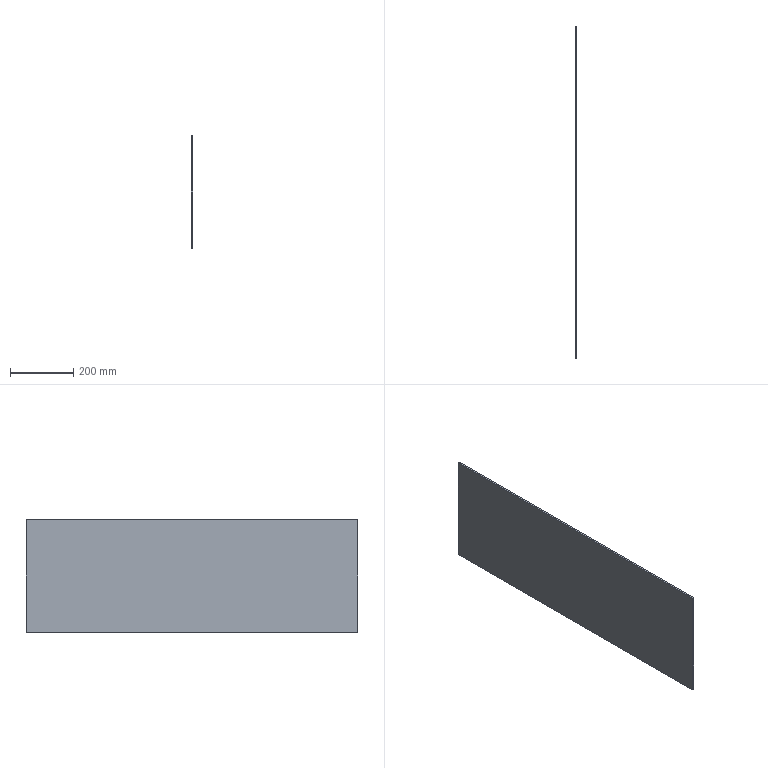Component | SolidWorks | BrownAcrylicPlate-5_BrownAcrylicPlate-2-2 | 1 solid | 6 faces | box 6 x 1049.15 x 355 mm | volume 2234689 mm3 | plane 6
STEP:
#1=CARTESIAN_POINT('',(-0.4379,39.232,-55.138));
#2=VERTEX_POINT('',#1);
#3=CARTESIAN_POINT('',(-0.4379,39.232,-69.114));
#4=VERTEX_POINT('',#3);
#5=CARTESIAN_POINT('',(-0.4379,39.232,-70.886));
#6=DIRECTION('',(-0.,0.,-1.));
#7=VECTOR('',#6,39.37);
#8=LINE('',#5,#7);
#9=EDGE_CURVE('',#2,#4,#8,.T.);
#10=ORIENTED_EDGE('',*,*,#9,.T.);
#11=CARTESIAN_POINT('',(-0.4379,80.537,-69.114));
#12=VERTEX_POINT('',#11);
#13=CARTESIAN_POINT('',(-0.4379,80.537,-69.114));
#14=DIRECTION('',(0.,1.,0.));
#15=VECTOR('',#14,39.37);
#16=LINE('',#13,#15);
#17=EDGE_CURVE('',#4,#12,#16,.T.);
#18=ORIENTED_EDGE('',*,*,#17,.T.);
#19=CARTESIAN_POINT('',(-0.4379,80.537,-55.138));
#20=VERTEX_POINT('',#19);
#21=CARTESIAN_POINT('',(-0.4379,80.537,-70.886));
#22=DIRECTION('',(0.,-0.,1.));
#23=VECTOR('',#22,39.37);
#24=LINE('',#21,#23);
#25=EDGE_CURVE('',#12,#20,#24,.T.);
#26=ORIENTED_EDGE('',*,*,#25,.T.);
#27=CARTESIAN_POINT('',(-0.4379,80.537,-55.138));
#28=DIRECTION('',(-0.,-1.,-0.));
#29=VECTOR('',#28,39.37);
#30=LINE('',#27,#29);
#31=EDGE_CURVE('',#20,#2,#30,.T.);
#32=ORIENTED_EDGE('',*,*,#31,.T.);
#33=EDGE_LOOP('',(#10,#18,#26,#32));
#34=FACE_OUTER_BOUND('',#33,.T.);
#35=CARTESIAN_POINT('',(-0.4379,69.711,-63.012));
#36=DIRECTION('',(1.,-0.,-0.));
#37=DIRECTION('',(0.,1.,0.));
#38=AXIS2_PLACEMENT_3D('',#35,#36,#37);
#39=PLANE('',#38);
#40=ADVANCED_FACE('',(#34),#39,.T.);
#41=CARTESIAN_POINT('',(-0.6741,39.232,-69.114));
#42=VERTEX_POINT('',#41);
#43=CARTESIAN_POINT('',(-0.6741,80.537,-69.114));
#44=VERTEX_POINT('',#43);
#45=CARTESIAN_POINT('',(-0.6741,69.711,-69.114));
#46=DIRECTION('',(0.,1.,0.));
#47=VECTOR('',#46,39.37);
#48=LINE('',#45,#47);
#49=EDGE_CURVE('',#42,#44,#48,.T.);
#50=ORIENTED_EDGE('',*,*,#49,.F.);
#51=CARTESIAN_POINT('',(-0.6741,39.232,-55.138));
#52=VERTEX_POINT('',#51);
#53=CARTESIAN_POINT('',(-0.6741,39.232,-63.012));
#54=DIRECTION('',(-0.,0.,-1.));
#55=VECTOR('',#54,39.37);
#56=LINE('',#53,#55);
#57=EDGE_CURVE('',#52,#42,#56,.T.);
#58=ORIENTED_EDGE('',*,*,#57,.F.);
#59=CARTESIAN_POINT('',(-0.6741,80.537,-55.138));
#60=VERTEX_POINT('',#59);
#61=CARTESIAN_POINT('',(-0.6741,69.711,-55.138));
#62=DIRECTION('',(-0.,-1.,-0.));
#63=VECTOR('',#62,39.37);
#64=LINE('',#61,#63);
#65=EDGE_CURVE('',#60,#52,#64,.T.);
#66=ORIENTED_EDGE('',*,*,#65,.F.);
#67=CARTESIAN_POINT('',(-0.6741,80.537,-63.012));
#68=DIRECTION('',(0.,-0.,1.));
#69=VECTOR('',#68,39.37);
#70=LINE('',#67,#69);
#71=EDGE_CURVE('',#44,#60,#70,.T.);
#72=ORIENTED_EDGE('',*,*,#71,.F.);
#73=EDGE_LOOP('',(#50,#58,#66,#72));
#74=FACE_OUTER_BOUND('',#73,.T.);
#75=CARTESIAN_POINT('',(-0.6741,69.711,-63.012));
#76=DIRECTION('',(1.,-0.,-0.));
#77=DIRECTION('',(0.,1.,0.));
#78=AXIS2_PLACEMENT_3D('',#75,#76,#77);
#79=PLANE('',#78);
#80=ADVANCED_FACE('',(#74),#79,.F.);
#81=ORIENTED_EDGE('',*,*,#71,.T.);
#82=CARTESIAN_POINT('',(-0.6741,80.537,-55.138));
#83=DIRECTION('',(1.,-0.,-0.));
#84=VECTOR('',#83,39.37);
#85=LINE('',#82,#84);
#86=EDGE_CURVE('',#60,#20,#85,.T.);
#87=ORIENTED_EDGE('',*,*,#86,.T.);
#88=ORIENTED_EDGE('',*,*,#25,.F.);
#89=CARTESIAN_POINT('',(-0.6741,80.537,-69.114));
#90=DIRECTION('',(1.,-0.,-0.));
#91=VECTOR('',#90,39.37);
#92=LINE('',#89,#91);
#93=EDGE_CURVE('',#44,#12,#92,.T.);
#94=ORIENTED_EDGE('',*,*,#93,.F.);
#95=EDGE_LOOP('',(#81,#87,#88,#94));
#96=FACE_OUTER_BOUND('',#95,.T.);
#97=CARTESIAN_POINT('',(-0.6741,80.537,-70.886));
#98=DIRECTION('',(-0.,-1.,-0.));
#99=DIRECTION('',(1.,-0.,-0.));
#100=AXIS2_PLACEMENT_3D('',#97,#98,#99);
#101=PLANE('',#100);
#102=ADVANCED_FACE('',(#96),#101,.F.);
#103=ORIENTED_EDGE('',*,*,#57,.T.);
#104=CARTESIAN_POINT('',(-0.6741,39.232,-69.114));
#105=DIRECTION('',(-1.,0.,0.));
#106=VECTOR('',#105,39.37);
#107=LINE('',#104,#106);
#108=EDGE_CURVE('',#4,#42,#107,.T.);
#109=ORIENTED_EDGE('',*,*,#108,.F.);
#110=ORIENTED_EDGE('',*,*,#9,.F.);
#111=CARTESIAN_POINT('',(-0.6741,39.232,-55.138));
#112=DIRECTION('',(1.,-0.,-0.));
#113=VECTOR('',#112,39.37);
#114=LINE('',#111,#113);
#115=EDGE_CURVE('',#52,#2,#114,.T.);
#116=ORIENTED_EDGE('',*,*,#115,.F.);
#117=EDGE_LOOP('',(#103,#109,#110,#116));
#118=FACE_OUTER_BOUND('',#117,.T.);
#119=CARTESIAN_POINT('',(-0.6741,39.232,-70.886));
#120=DIRECTION('',(0.,1.,0.));
#121=DIRECTION('',(-1.,0.,0.));
#122=AXIS2_PLACEMENT_3D('',#119,#120,#121);
#123=PLANE('',#122);
#124=ADVANCED_FACE('',(#118),#123,.F.);
#125=ORIENTED_EDGE('',*,*,#65,.T.);
#126=ORIENTED_EDGE('',*,*,#115,.T.);
#127=ORIENTED_EDGE('',*,*,#31,.F.);
#128=ORIENTED_EDGE('',*,*,#86,.F.);
#129=EDGE_LOOP('',(#125,#126,#127,#128));
#130=FACE_OUTER_BOUND('',#129,.T.);
#131=CARTESIAN_POINT('',(-0.6741,80.537,-55.138));
#132=DIRECTION('',(-0.,0.,-1.));
#133=DIRECTION('',(-0.,-1.,-0.));
#134=AXIS2_PLACEMENT_3D('',#131,#132,#133);
#135=PLANE('',#134);
#136=ADVANCED_FACE('',(#130),#135,.F.);
#137=ORIENTED_EDGE('',*,*,#17,.F.);
#138=ORIENTED_EDGE('',*,*,#108,.T.);
#139=ORIENTED_EDGE('',*,*,#49,.T.);
#140=ORIENTED_EDGE('',*,*,#93,.T.);
#141=EDGE_LOOP('',(#137,#138,#139,#140));
#142=FACE_OUTER_BOUND('',#141,.T.);
#143=CARTESIAN_POINT('',(-0.6741,80.537,-69.114));
#144=DIRECTION('',(0.,-0.,1.));
#145=DIRECTION('',(0.,1.,0.));
#146=AXIS2_PLACEMENT_3D('',#143,#144,#145);
#147=PLANE('',#146);
#148=ADVANCED_FACE('',(#142),#147,.F.);
#149=CLOSED_SHELL('',(#40,#80,#102,#124,#136,#148));
#150=MANIFOLD_SOLID_BREP('',#149);
#151=CARTESIAN_POINT('',(0.,0.,0.));
#152=DIRECTION('',(0.,0.,1.));
#153=DIRECTION('',(1.,0.,0.));
#154=AXIS2_PLACEMENT_3D('',#151,#152,#153);
#155=(LENGTH_UNIT()NAMED_UNIT(*)SI_UNIT($,.METRE.));
#156=LENGTH_MEASURE_WITH_UNIT(LENGTH_MEASURE(0.0254),#155);
#157=DIMENSIONAL_EXPONENTS(1.,0.,0.,0.,0.,0.,0.);
#158=(CONVERSION_BASED_UNIT('',#156)LENGTH_UNIT()NAMED_UNIT(#157));
#159=UNCERTAINTY_MEASURE_WITH_UNIT(LENGTH_MEASURE(0.00001),#158,'','');
#160=(NAMED_UNIT(*)PLANE_ANGLE_UNIT()SI_UNIT($,.RADIAN.));
#161=(NAMED_UNIT(*)SI_UNIT($,.STERADIAN.)SOLID_ANGLE_UNIT());
#162=(GEOMETRIC_REPRESENTATION_CONTEXT(3)GLOBAL_UNCERTAINTY_ASSIGNED_CONTEXT((#159))GLOBAL_UNIT_ASSIGNED_CONTEXT((#158,#160,#161))REPRESENTATION_CONTEXT('',''));
#163=ADVANCED_BREP_SHAPE_REPRESENTATION('',(#150,#154),#162);
#164=COLOUR_RGB('',0.7922,0.8196,0.9333);
#165=FILL_AREA_STYLE_COLOUR('',#164);
#166=FILL_AREA_STYLE('',(#165));
#167=SURFACE_STYLE_FILL_AREA(#166);
#168=SURFACE_SIDE_STYLE('',(#167));
#169=SURFACE_STYLE_USAGE(.BOTH.,#168);
#170=PRESENTATION_STYLE_ASSIGNMENT((#169));
#171=STYLED_ITEM('',(#170),#150);
#172=(LENGTH_UNIT()NAMED_UNIT(*)SI_UNIT($,.METRE.));
#173=LENGTH_MEASURE_WITH_UNIT(LENGTH_MEASURE(0.0254),#172);
#174=DIMENSIONAL_EXPONENTS(1.,0.,0.,0.,0.,0.,0.);
#175=(CONVERSION_BASED_UNIT('',#173)LENGTH_UNIT()NAMED_UNIT(#174));
#176=UNCERTAINTY_MEASURE_WITH_UNIT(LENGTH_MEASURE(0.00001),#175,'','');
#177=(NAMED_UNIT(*)PLANE_ANGLE_UNIT()SI_UNIT($,.RADIAN.));
#178=(NAMED_UNIT(*)SI_UNIT($,.STERADIAN.)SOLID_ANGLE_UNIT());
#179=(GEOMETRIC_REPRESENTATION_CONTEXT(3)GLOBAL_UNCERTAINTY_ASSIGNED_CONTEXT((#176))GLOBAL_UNIT_ASSIGNED_CONTEXT((#175,#177,#178))REPRESENTATION_CONTEXT('',''));
#180=MECHANICAL_DESIGN_GEOMETRIC_PRESENTATION_REPRESENTATION('',(#171),#179);
#181=PRESENTATION_LAYER_ASSIGNMENT('','',(#171));